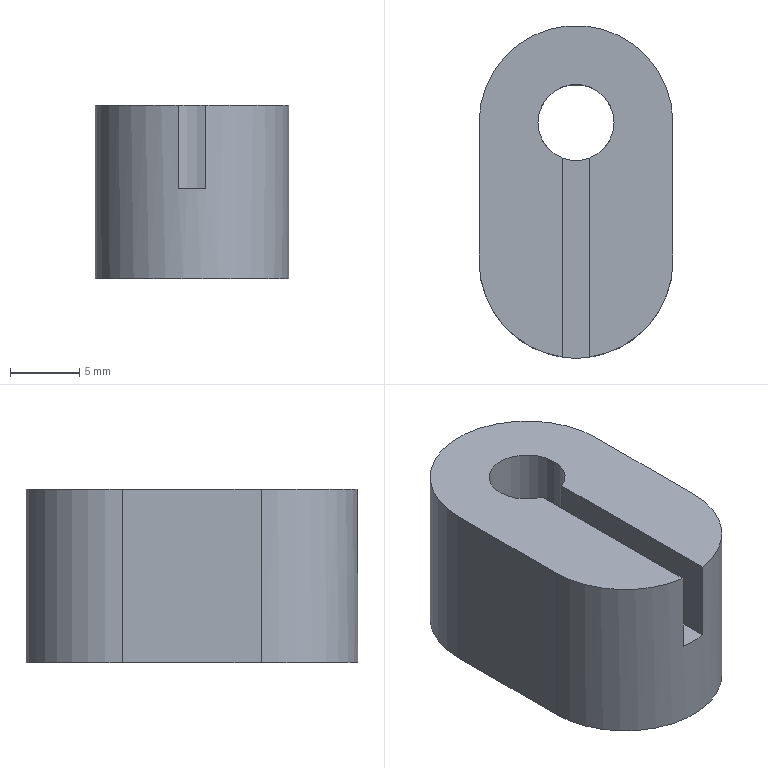Component | SolidWorks | CLS-MechanismAccessory2-1 | 1 solid | 11 faces | box 14 x 24 x 12.5 mm | volume 3206 mm3 | plane 7 | cylinder 4 | commonest cylinder face diameters 5.5 x2 14 x2
build123d program:
from build123d import *

# Parameters (mm, degrees)
SKETCH4_R           = 2.75
BOSS_EXTRUDE1_DEPTH = 12.5
SKETCH5_W           = 2
SKETCH5_H           = 30
CUT_EXTRUDE1_DEPTH  = 6


with BuildPart() as part:
    # Sketch4 → Boss-Extrude1 (new body)
    with BuildSketch(Plane.XY):
        with BuildLine():
            Line((7, 5), (7, -5))
            ThreePointArc((7, -5), (0, -12), (-7, -5))
            Line((-7, -5), (-7, 5))
            ThreePointArc((-7, 5), (0, 12), (7, 5))
        make_face()
        with Locations((0, 5)):
            Circle(SKETCH4_R, mode=Mode.SUBTRACT)
    extrude(amount=BOSS_EXTRUDE1_DEPTH)

    # Sketch5 → Cut-Extrude1 (cut)
    with BuildSketch(Plane.XY):
        with Locations((0, -12)):
            Rectangle(SKETCH5_W, SKETCH5_H)
    extrude(amount=CUT_EXTRUDE1_DEPTH, mode=Mode.SUBTRACT)


solid = part.part

# Placed as in the assembly
solid = solid.moved(Location((-24.526, 12.192, -5.001), (-180, 0, 180)))
STEP:
#1=COLOUR_RGB('',0.7922,0.8196,0.9333);
#2=FILL_AREA_STYLE_COLOUR('',#1);
#3=FILL_AREA_STYLE('',(#2));
#4=SURFACE_STYLE_FILL_AREA(#3);
#5=SURFACE_SIDE_STYLE('',(#4));
#6=SURFACE_STYLE_USAGE(.BOTH.,#5);
#7=PRESENTATION_STYLE_ASSIGNMENT((#6));
#8=CARTESIAN_POINT('',(-0.8573,0.6769,-0.689));
#9=VERTEX_POINT('',#8);
#10=CARTESIAN_POINT('',(-1.074,0.6769,-0.689));
#11=VERTEX_POINT('',#10);
#12=CARTESIAN_POINT('',(-0.9656,0.6769,-0.689));
#13=DIRECTION('',(-0.,0.,-1.));
#14=DIRECTION('',(-1.,0.,0.));
#15=AXIS2_PLACEMENT_3D('',#12,#13,#14);
#16=CIRCLE('',#15,0.1083);
#17=EDGE_CURVE('',#9,#11,#16,.T.);
#18=ORIENTED_EDGE('',*,*,#17,.T.);
#19=CARTESIAN_POINT('',(-1.074,0.6769,-0.1969));
#20=VERTEX_POINT('',#19);
#21=CARTESIAN_POINT('',(-1.074,0.6769,-0.689));
#22=DIRECTION('',(0.,-0.,1.));
#23=VECTOR('',#22,39.37);
#24=LINE('',#21,#23);
#25=EDGE_CURVE('',#11,#20,#24,.T.);
#26=ORIENTED_EDGE('',*,*,#25,.T.);
#27=CARTESIAN_POINT('',(-1.005,0.576,-0.1969));
#28=VERTEX_POINT('',#27);
#29=CARTESIAN_POINT('',(-0.9656,0.6769,-0.1969));
#30=DIRECTION('',(-0.,0.,-1.));
#31=DIRECTION('',(-1.,0.,0.));
#32=AXIS2_PLACEMENT_3D('',#29,#30,#31);
#33=CIRCLE('',#32,0.1083);
#34=EDGE_CURVE('',#28,#20,#33,.T.);
#35=ORIENTED_EDGE('',*,*,#34,.F.);
#36=CARTESIAN_POINT('',(-1.005,0.576,-0.4331));
#37=VERTEX_POINT('',#36);
#38=CARTESIAN_POINT('',(-1.005,0.576,-0.689));
#39=DIRECTION('',(-0.,0.,-1.));
#40=VECTOR('',#39,39.37);
#41=LINE('',#38,#40);
#42=EDGE_CURVE('',#28,#37,#41,.T.);
#43=ORIENTED_EDGE('',*,*,#42,.T.);
#44=CARTESIAN_POINT('',(-0.9262,0.576,-0.4331));
#45=VERTEX_POINT('',#44);
#46=CARTESIAN_POINT('',(-0.9656,0.6769,-0.4331));
#47=DIRECTION('',(0.,-0.,1.));
#48=DIRECTION('',(1.,0.,-0.));
#49=AXIS2_PLACEMENT_3D('',#46,#47,#48);
#50=CIRCLE('',#49,0.1083);
#51=EDGE_CURVE('',#37,#45,#50,.T.);
#52=ORIENTED_EDGE('',*,*,#51,.T.);
#53=CARTESIAN_POINT('',(-0.9262,0.576,-0.1969));
#54=VERTEX_POINT('',#53);
#55=CARTESIAN_POINT('',(-0.9262,0.576,-0.689));
#56=DIRECTION('',(0.,-0.,1.));
#57=VECTOR('',#56,39.37);
#58=LINE('',#55,#57);
#59=EDGE_CURVE('',#45,#54,#58,.T.);
#60=ORIENTED_EDGE('',*,*,#59,.T.);
#61=CARTESIAN_POINT('',(-0.8573,0.6769,-0.1969));
#62=VERTEX_POINT('',#61);
#63=CARTESIAN_POINT('',(-0.9656,0.6769,-0.1969));
#64=DIRECTION('',(-0.,0.,-1.));
#65=DIRECTION('',(-1.,0.,0.));
#66=AXIS2_PLACEMENT_3D('',#63,#64,#65);
#67=CIRCLE('',#66,0.1083);
#68=EDGE_CURVE('',#62,#54,#67,.T.);
#69=ORIENTED_EDGE('',*,*,#68,.F.);
#70=CARTESIAN_POINT('',(-0.8573,0.6769,-0.689));
#71=DIRECTION('',(0.,-0.,1.));
#72=VECTOR('',#71,39.37);
#73=LINE('',#70,#72);
#74=EDGE_CURVE('',#9,#62,#73,.T.);
#75=ORIENTED_EDGE('',*,*,#74,.F.);
#76=EDGE_LOOP('',(#18,#26,#35,#43,#52,#60,#69,#75));
#77=FACE_OUTER_BOUND('',#76,.T.);
#78=CARTESIAN_POINT('',(-0.9656,0.6769,-0.689));
#79=DIRECTION('',(0.,-0.,1.));
#80=DIRECTION('',(1.,0.,0.));
#81=AXIS2_PLACEMENT_3D('',#78,#79,#80);
#82=CYLINDRICAL_SURFACE('',#81,0.1083);
#83=ADVANCED_FACE('',(#77),#82,.F.);
#84=CARTESIAN_POINT('',(-1.005,0.01039,-0.1969));
#85=VERTEX_POINT('',#84);
#86=CARTESIAN_POINT('',(-1.005,-0.583,-0.1969));
#87=DIRECTION('',(0.,1.,-0.));
#88=VECTOR('',#87,39.37);
#89=LINE('',#86,#88);
#90=EDGE_CURVE('',#85,#28,#89,.T.);
#91=ORIENTED_EDGE('',*,*,#90,.T.);
#92=ORIENTED_EDGE('',*,*,#34,.T.);
#93=CARTESIAN_POINT('',(-0.9656,0.6769,-0.1969));
#94=DIRECTION('',(-0.,0.,-1.));
#95=DIRECTION('',(-1.,0.,0.));
#96=AXIS2_PLACEMENT_3D('',#93,#94,#95);
#97=CIRCLE('',#96,0.1083);
#98=EDGE_CURVE('',#20,#62,#97,.T.);
#99=ORIENTED_EDGE('',*,*,#98,.T.);
#100=ORIENTED_EDGE('',*,*,#68,.T.);
#101=CARTESIAN_POINT('',(-0.9262,0.01039,-0.1969));
#102=VERTEX_POINT('',#101);
#103=CARTESIAN_POINT('',(-0.9262,-0.583,-0.1969));
#104=DIRECTION('',(-0.,-1.,0.));
#105=VECTOR('',#104,39.37);
#106=LINE('',#103,#105);
#107=EDGE_CURVE('',#54,#102,#106,.T.);
#108=ORIENTED_EDGE('',*,*,#107,.T.);
#109=CARTESIAN_POINT('',(-0.69,0.2832,-0.1969));
#110=VERTEX_POINT('',#109);
#111=CARTESIAN_POINT('',(-0.9656,0.2832,-0.1969));
#112=DIRECTION('',(-0.,0.,-1.));
#113=DIRECTION('',(-1.,0.,0.));
#114=AXIS2_PLACEMENT_3D('',#111,#112,#113);
#115=CIRCLE('',#114,0.2756);
#116=EDGE_CURVE('',#110,#102,#115,.T.);
#117=ORIENTED_EDGE('',*,*,#116,.F.);
#118=CARTESIAN_POINT('',(-0.69,0.6769,-0.1969));
#119=VERTEX_POINT('',#118);
#120=CARTESIAN_POINT('',(-0.69,0.6769,-0.1969));
#121=DIRECTION('',(-0.,-1.,0.));
#122=VECTOR('',#121,39.37);
#123=LINE('',#120,#122);
#124=EDGE_CURVE('',#119,#110,#123,.T.);
#125=ORIENTED_EDGE('',*,*,#124,.F.);
#126=CARTESIAN_POINT('',(-1.241,0.6769,-0.1969));
#127=VERTEX_POINT('',#126);
#128=CARTESIAN_POINT('',(-0.9656,0.6769,-0.1969));
#129=DIRECTION('',(-0.,0.,-1.));
#130=DIRECTION('',(-1.,0.,0.));
#131=AXIS2_PLACEMENT_3D('',#128,#129,#130);
#132=CIRCLE('',#131,0.2756);
#133=EDGE_CURVE('',#127,#119,#132,.T.);
#134=ORIENTED_EDGE('',*,*,#133,.F.);
#135=CARTESIAN_POINT('',(-1.241,0.2832,-0.1969));
#136=VERTEX_POINT('',#135);
#137=CARTESIAN_POINT('',(-1.241,0.6769,-0.1969));
#138=DIRECTION('',(0.,1.,-0.));
#139=VECTOR('',#138,39.37);
#140=LINE('',#137,#139);
#141=EDGE_CURVE('',#136,#127,#140,.T.);
#142=ORIENTED_EDGE('',*,*,#141,.F.);
#143=CARTESIAN_POINT('',(-0.9656,0.2832,-0.1969));
#144=DIRECTION('',(-0.,0.,-1.));
#145=DIRECTION('',(-1.,0.,0.));
#146=AXIS2_PLACEMENT_3D('',#143,#144,#145);
#147=CIRCLE('',#146,0.2756);
#148=EDGE_CURVE('',#85,#136,#147,.T.);
#149=ORIENTED_EDGE('',*,*,#148,.F.);
#150=EDGE_LOOP('',(#91,#92,#99,#100,#108,#117,#125,#134,#142,#149));
#151=FACE_OUTER_BOUND('',#150,.T.);
#152=CARTESIAN_POINT('',(-0.9656,0.6769,-0.1969));
#153=DIRECTION('',(-0.,0.,-1.));
#154=DIRECTION('',(-1.,0.,0.));
#155=AXIS2_PLACEMENT_3D('',#152,#153,#154);
#156=PLANE('',#155);
#157=ADVANCED_FACE('',(#151),#156,.F.);
#158=CARTESIAN_POINT('',(-1.005,0.01039,-0.4331));
#159=VERTEX_POINT('',#158);
#160=CARTESIAN_POINT('',(-1.005,0.01039,-0.689));
#161=DIRECTION('',(-0.,0.,-1.));
#162=VECTOR('',#161,39.37);
#163=LINE('',#160,#162);
#164=EDGE_CURVE('',#85,#159,#163,.T.);
#165=ORIENTED_EDGE('',*,*,#164,.F.);
#166=ORIENTED_EDGE('',*,*,#148,.T.);
#167=CARTESIAN_POINT('',(-1.241,0.2832,-0.689));
#168=VERTEX_POINT('',#167);
#169=CARTESIAN_POINT('',(-1.241,0.2832,-0.689));
#170=DIRECTION('',(0.,-0.,1.));
#171=VECTOR('',#170,39.37);
#172=LINE('',#169,#171);
#173=EDGE_CURVE('',#168,#136,#172,.T.);
#174=ORIENTED_EDGE('',*,*,#173,.F.);
#175=CARTESIAN_POINT('',(-0.69,0.2832,-0.689));
#176=VERTEX_POINT('',#175);
#177=CARTESIAN_POINT('',(-0.9656,0.2832,-0.689));
#178=DIRECTION('',(-0.,0.,-1.));
#179=DIRECTION('',(-1.,0.,0.));
#180=AXIS2_PLACEMENT_3D('',#177,#178,#179);
#181=CIRCLE('',#180,0.2756);
#182=EDGE_CURVE('',#176,#168,#181,.T.);
#183=ORIENTED_EDGE('',*,*,#182,.F.);
#184=CARTESIAN_POINT('',(-0.69,0.2832,-0.689));
#185=DIRECTION('',(0.,-0.,1.));
#186=VECTOR('',#185,39.37);
#187=LINE('',#184,#186);
#188=EDGE_CURVE('',#176,#110,#187,.T.);
#189=ORIENTED_EDGE('',*,*,#188,.T.);
#190=ORIENTED_EDGE('',*,*,#116,.T.);
#191=CARTESIAN_POINT('',(-0.9262,0.01039,-0.4331));
#192=VERTEX_POINT('',#191);
#193=CARTESIAN_POINT('',(-0.9262,0.01039,-0.689));
#194=DIRECTION('',(0.,-0.,1.));
#195=VECTOR('',#194,39.37);
#196=LINE('',#193,#195);
#197=EDGE_CURVE('',#192,#102,#196,.T.);
#198=ORIENTED_EDGE('',*,*,#197,.F.);
#199=CARTESIAN_POINT('',(-0.9656,0.2832,-0.4331));
#200=DIRECTION('',(0.,-0.,1.));
#201=DIRECTION('',(1.,-0.,-0.));
#202=AXIS2_PLACEMENT_3D('',#199,#200,#201);
#203=CIRCLE('',#202,0.2756);
#204=EDGE_CURVE('',#159,#192,#203,.T.);
#205=ORIENTED_EDGE('',*,*,#204,.F.);
#206=EDGE_LOOP('',(#165,#166,#174,#183,#189,#190,#198,#205));
#207=FACE_OUTER_BOUND('',#206,.T.);
#208=CARTESIAN_POINT('',(-0.9656,0.2832,-0.689));
#209=DIRECTION('',(0.,-0.,1.));
#210=DIRECTION('',(1.,-0.,-0.));
#211=AXIS2_PLACEMENT_3D('',#208,#209,#210);
#212=CYLINDRICAL_SURFACE('',#211,0.2756);
#213=ADVANCED_FACE('',(#207),#212,.T.);
#214=ORIENTED_EDGE('',*,*,#25,.F.);
#215=CARTESIAN_POINT('',(-0.9656,0.6769,-0.689));
#216=DIRECTION('',(-0.,0.,-1.));
#217=DIRECTION('',(-1.,0.,0.));
#218=AXIS2_PLACEMENT_3D('',#215,#216,#217);
#219=CIRCLE('',#218,0.1083);
#220=EDGE_CURVE('',#11,#9,#219,.T.);
#221=ORIENTED_EDGE('',*,*,#220,.T.);
#222=ORIENTED_EDGE('',*,*,#74,.T.);
#223=ORIENTED_EDGE('',*,*,#98,.F.);
#224=EDGE_LOOP('',(#214,#221,#222,#223));
#225=FACE_OUTER_BOUND('',#224,.T.);
#226=CARTESIAN_POINT('',(-0.9656,0.6769,-0.689));
#227=DIRECTION('',(0.,-0.,1.));
#228=DIRECTION('',(1.,0.,0.));
#229=AXIS2_PLACEMENT_3D('',#226,#227,#228);
#230=CYLINDRICAL_SURFACE('',#229,0.1083);
#231=ADVANCED_FACE('',(#225),#230,.F.);
#232=CARTESIAN_POINT('',(-1.241,0.6769,-0.689));
#233=VERTEX_POINT('',#232);
#234=CARTESIAN_POINT('',(-0.69,0.6769,-0.689));
#235=VERTEX_POINT('',#234);
#236=CARTESIAN_POINT('',(-0.9656,0.6769,-0.689));
#237=DIRECTION('',(-0.,0.,-1.));
#238=DIRECTION('',(-1.,0.,0.));
#239=AXIS2_PLACEMENT_3D('',#236,#237,#238);
#240=CIRCLE('',#239,0.2756);
#241=EDGE_CURVE('',#233,#235,#240,.T.);
#242=ORIENTED_EDGE('',*,*,#241,.T.);
#243=CARTESIAN_POINT('',(-0.69,0.6769,-0.689));
#244=DIRECTION('',(-0.,-1.,0.));
#245=VECTOR('',#244,39.37);
#246=LINE('',#243,#245);
#247=EDGE_CURVE('',#235,#176,#246,.T.);
#248=ORIENTED_EDGE('',*,*,#247,.T.);
#249=ORIENTED_EDGE('',*,*,#182,.T.);
#250=CARTESIAN_POINT('',(-1.241,0.6769,-0.689));
#251=DIRECTION('',(0.,1.,-0.));
#252=VECTOR('',#251,39.37);
#253=LINE('',#250,#252);
#254=EDGE_CURVE('',#168,#233,#253,.T.);
#255=ORIENTED_EDGE('',*,*,#254,.T.);
#256=EDGE_LOOP('',(#242,#248,#249,#255));
#257=FACE_OUTER_BOUND('',#256,.T.);
#258=ORIENTED_EDGE('',*,*,#17,.F.);
#259=ORIENTED_EDGE('',*,*,#220,.F.);
#260=EDGE_LOOP('',(#258,#259));
#261=FACE_BOUND('',#260,.T.);
#262=CARTESIAN_POINT('',(-0.9656,0.6769,-0.689));
#263=DIRECTION('',(-0.,0.,-1.));
#264=DIRECTION('',(-1.,0.,0.));
#265=AXIS2_PLACEMENT_3D('',#262,#263,#264);
#266=PLANE('',#265);
#267=ADVANCED_FACE('',(#257,#261),#266,.T.);
#268=ORIENTED_EDGE('',*,*,#133,.T.);
#269=CARTESIAN_POINT('',(-0.69,0.6769,-0.689));
#270=DIRECTION('',(0.,-0.,1.));
#271=VECTOR('',#270,39.37);
#272=LINE('',#269,#271);
#273=EDGE_CURVE('',#235,#119,#272,.T.);
#274=ORIENTED_EDGE('',*,*,#273,.F.);
#275=ORIENTED_EDGE('',*,*,#241,.F.);
#276=CARTESIAN_POINT('',(-1.241,0.6769,-0.689));
#277=DIRECTION('',(0.,-0.,1.));
#278=VECTOR('',#277,39.37);
#279=LINE('',#276,#278);
#280=EDGE_CURVE('',#233,#127,#279,.T.);
#281=ORIENTED_EDGE('',*,*,#280,.T.);
#282=EDGE_LOOP('',(#268,#274,#275,#281));
#283=FACE_OUTER_BOUND('',#282,.T.);
#284=CARTESIAN_POINT('',(-0.9656,0.6769,-0.689));
#285=DIRECTION('',(0.,-0.,1.));
#286=DIRECTION('',(1.,0.,-0.));
#287=AXIS2_PLACEMENT_3D('',#284,#285,#286);
#288=CYLINDRICAL_SURFACE('',#287,0.2756);
#289=ADVANCED_FACE('',(#283),#288,.T.);
#290=ORIENTED_EDGE('',*,*,#124,.T.);
#291=ORIENTED_EDGE('',*,*,#188,.F.);
#292=ORIENTED_EDGE('',*,*,#247,.F.);
#293=ORIENTED_EDGE('',*,*,#273,.T.);
#294=EDGE_LOOP('',(#290,#291,#292,#293));
#295=FACE_OUTER_BOUND('',#294,.T.);
#296=CARTESIAN_POINT('',(-0.69,0.6769,-0.689));
#297=DIRECTION('',(-1.,0.,0.));
#298=DIRECTION('',(0.,-0.,1.));
#299=AXIS2_PLACEMENT_3D('',#296,#297,#298);
#300=PLANE('',#299);
#301=ADVANCED_FACE('',(#295),#300,.F.);
#302=ORIENTED_EDGE('',*,*,#141,.T.);
#303=ORIENTED_EDGE('',*,*,#280,.F.);
#304=ORIENTED_EDGE('',*,*,#254,.F.);
#305=ORIENTED_EDGE('',*,*,#173,.T.);
#306=EDGE_LOOP('',(#302,#303,#304,#305));
#307=FACE_OUTER_BOUND('',#306,.T.);
#308=CARTESIAN_POINT('',(-1.241,0.6769,-0.689));
#309=DIRECTION('',(1.,-0.,-0.));
#310=DIRECTION('',(-0.,-1.,0.));
#311=AXIS2_PLACEMENT_3D('',#308,#309,#310);
#312=PLANE('',#311);
#313=ADVANCED_FACE('',(#307),#312,.F.);
#314=ORIENTED_EDGE('',*,*,#164,.T.);
#315=CARTESIAN_POINT('',(-1.005,-0.583,-0.4331));
#316=DIRECTION('',(0.,1.,-0.));
#317=VECTOR('',#316,39.37);
#318=LINE('',#315,#317);
#319=EDGE_CURVE('',#159,#37,#318,.T.);
#320=ORIENTED_EDGE('',*,*,#319,.T.);
#321=ORIENTED_EDGE('',*,*,#42,.F.);
#322=ORIENTED_EDGE('',*,*,#90,.F.);
#323=EDGE_LOOP('',(#314,#320,#321,#322));
#324=FACE_OUTER_BOUND('',#323,.T.);
#325=CARTESIAN_POINT('',(-1.005,-0.583,-0.4331));
#326=DIRECTION('',(1.,-0.,-0.));
#327=DIRECTION('',(-0.,0.,-1.));
#328=AXIS2_PLACEMENT_3D('',#325,#326,#327);
#329=PLANE('',#328);
#330=ADVANCED_FACE('',(#324),#329,.T.);
#331=ORIENTED_EDGE('',*,*,#197,.T.);
#332=ORIENTED_EDGE('',*,*,#107,.F.);
#333=ORIENTED_EDGE('',*,*,#59,.F.);
#334=CARTESIAN_POINT('',(-0.9262,-0.583,-0.4331));
#335=DIRECTION('',(-0.,-1.,0.));
#336=VECTOR('',#335,39.37);
#337=LINE('',#334,#336);
#338=EDGE_CURVE('',#45,#192,#337,.T.);
#339=ORIENTED_EDGE('',*,*,#338,.T.);
#340=EDGE_LOOP('',(#331,#332,#333,#339));
#341=FACE_OUTER_BOUND('',#340,.T.);
#342=CARTESIAN_POINT('',(-0.9262,-0.583,-0.4331));
#343=DIRECTION('',(-1.,0.,0.));
#344=DIRECTION('',(0.,-0.,1.));
#345=AXIS2_PLACEMENT_3D('',#342,#343,#344);
#346=PLANE('',#345);
#347=ADVANCED_FACE('',(#341),#346,.T.);
#348=ORIENTED_EDGE('',*,*,#204,.T.);
#349=ORIENTED_EDGE('',*,*,#338,.F.);
#350=ORIENTED_EDGE('',*,*,#51,.F.);
#351=ORIENTED_EDGE('',*,*,#319,.F.);
#352=EDGE_LOOP('',(#348,#349,#350,#351));
#353=FACE_OUTER_BOUND('',#352,.T.);
#354=CARTESIAN_POINT('',(-1.005,0.5981,-0.4331));
#355=DIRECTION('',(0.,-0.,1.));
#356=DIRECTION('',(1.,-0.,-0.));
#357=AXIS2_PLACEMENT_3D('',#354,#355,#356);
#358=PLANE('',#357);
#359=ADVANCED_FACE('',(#353),#358,.T.);
#360=CLOSED_SHELL('',(#83,#157,#213,#231,#267,#289,#301,#313,#330,#347,#359));
#361=MANIFOLD_SOLID_BREP('',#360);
#362=STYLED_ITEM('',(#7),#361);
#363=(LENGTH_UNIT()NAMED_UNIT(*)SI_UNIT($,.METRE.));
#364=LENGTH_MEASURE_WITH_UNIT(LENGTH_MEASURE(0.0254),#363);
#365=DIMENSIONAL_EXPONENTS(1.,0.,0.,0.,0.,0.,0.);
#366=(CONVERSION_BASED_UNIT('',#364)LENGTH_UNIT()NAMED_UNIT(#365));
#367=UNCERTAINTY_MEASURE_WITH_UNIT(LENGTH_MEASURE(0.00001),#366,'','');
#368=(NAMED_UNIT(*)PLANE_ANGLE_UNIT()SI_UNIT($,.RADIAN.));
#369=(NAMED_UNIT(*)SI_UNIT($,.STERADIAN.)SOLID_ANGLE_UNIT());
#370=(GEOMETRIC_REPRESENTATION_CONTEXT(3)GLOBAL_UNCERTAINTY_ASSIGNED_CONTEXT((#367))GLOBAL_UNIT_ASSIGNED_CONTEXT((#366,#368,#369))REPRESENTATION_CONTEXT('',''));
#371=MECHANICAL_DESIGN_GEOMETRIC_PRESENTATION_REPRESENTATION('',(#362),#370);
#372=PRESENTATION_LAYER_ASSIGNMENT('','',(#362));
#373=CARTESIAN_POINT('',(0.,0.,0.));
#374=DIRECTION('',(0.,0.,1.));
#375=DIRECTION('',(1.,0.,0.));
#376=AXIS2_PLACEMENT_3D('',#373,#374,#375);
#377=(LENGTH_UNIT()NAMED_UNIT(*)SI_UNIT($,.METRE.));
#378=LENGTH_MEASURE_WITH_UNIT(LENGTH_MEASURE(0.0254),#377);
#379=DIMENSIONAL_EXPONENTS(1.,0.,0.,0.,0.,0.,0.);
#380=(CONVERSION_BASED_UNIT('',#378)LENGTH_UNIT()NAMED_UNIT(#379));
#381=UNCERTAINTY_MEASURE_WITH_UNIT(LENGTH_MEASURE(0.00001),#380,'','');
#382=(NAMED_UNIT(*)PLANE_ANGLE_UNIT()SI_UNIT($,.RADIAN.));
#383=(NAMED_UNIT(*)SI_UNIT($,.STERADIAN.)SOLID_ANGLE_UNIT());
#384=(GEOMETRIC_REPRESENTATION_CONTEXT(3)GLOBAL_UNCERTAINTY_ASSIGNED_CONTEXT((#381))GLOBAL_UNIT_ASSIGNED_CONTEXT((#380,#382,#383))REPRESENTATION_CONTEXT('',''));
#385=ADVANCED_BREP_SHAPE_REPRESENTATION('',(#361,#376),#384);